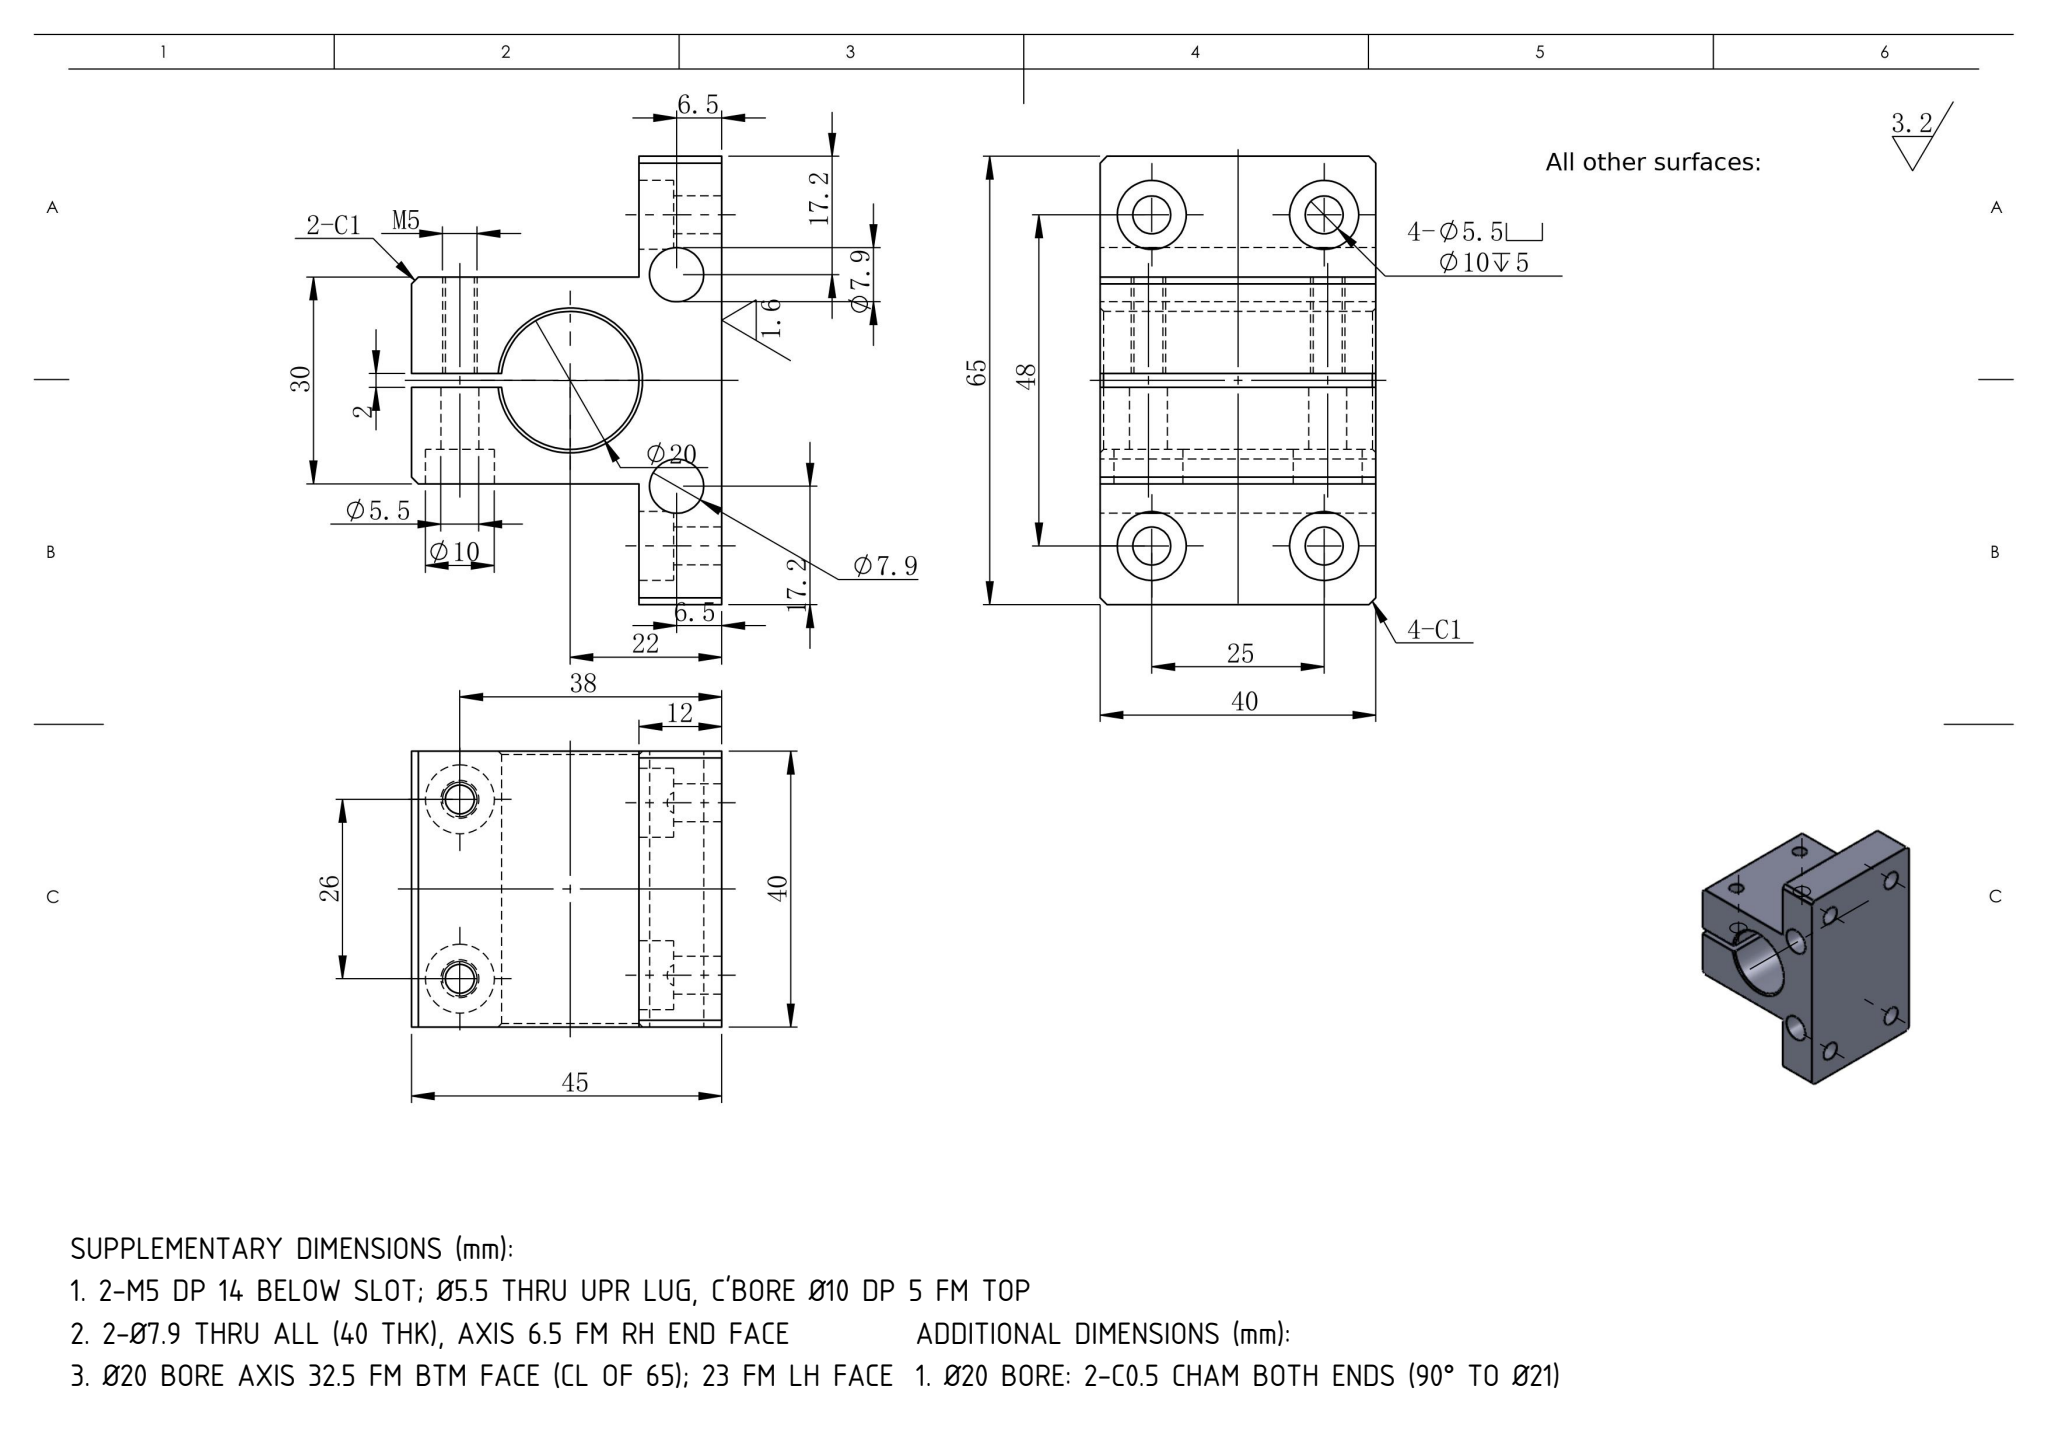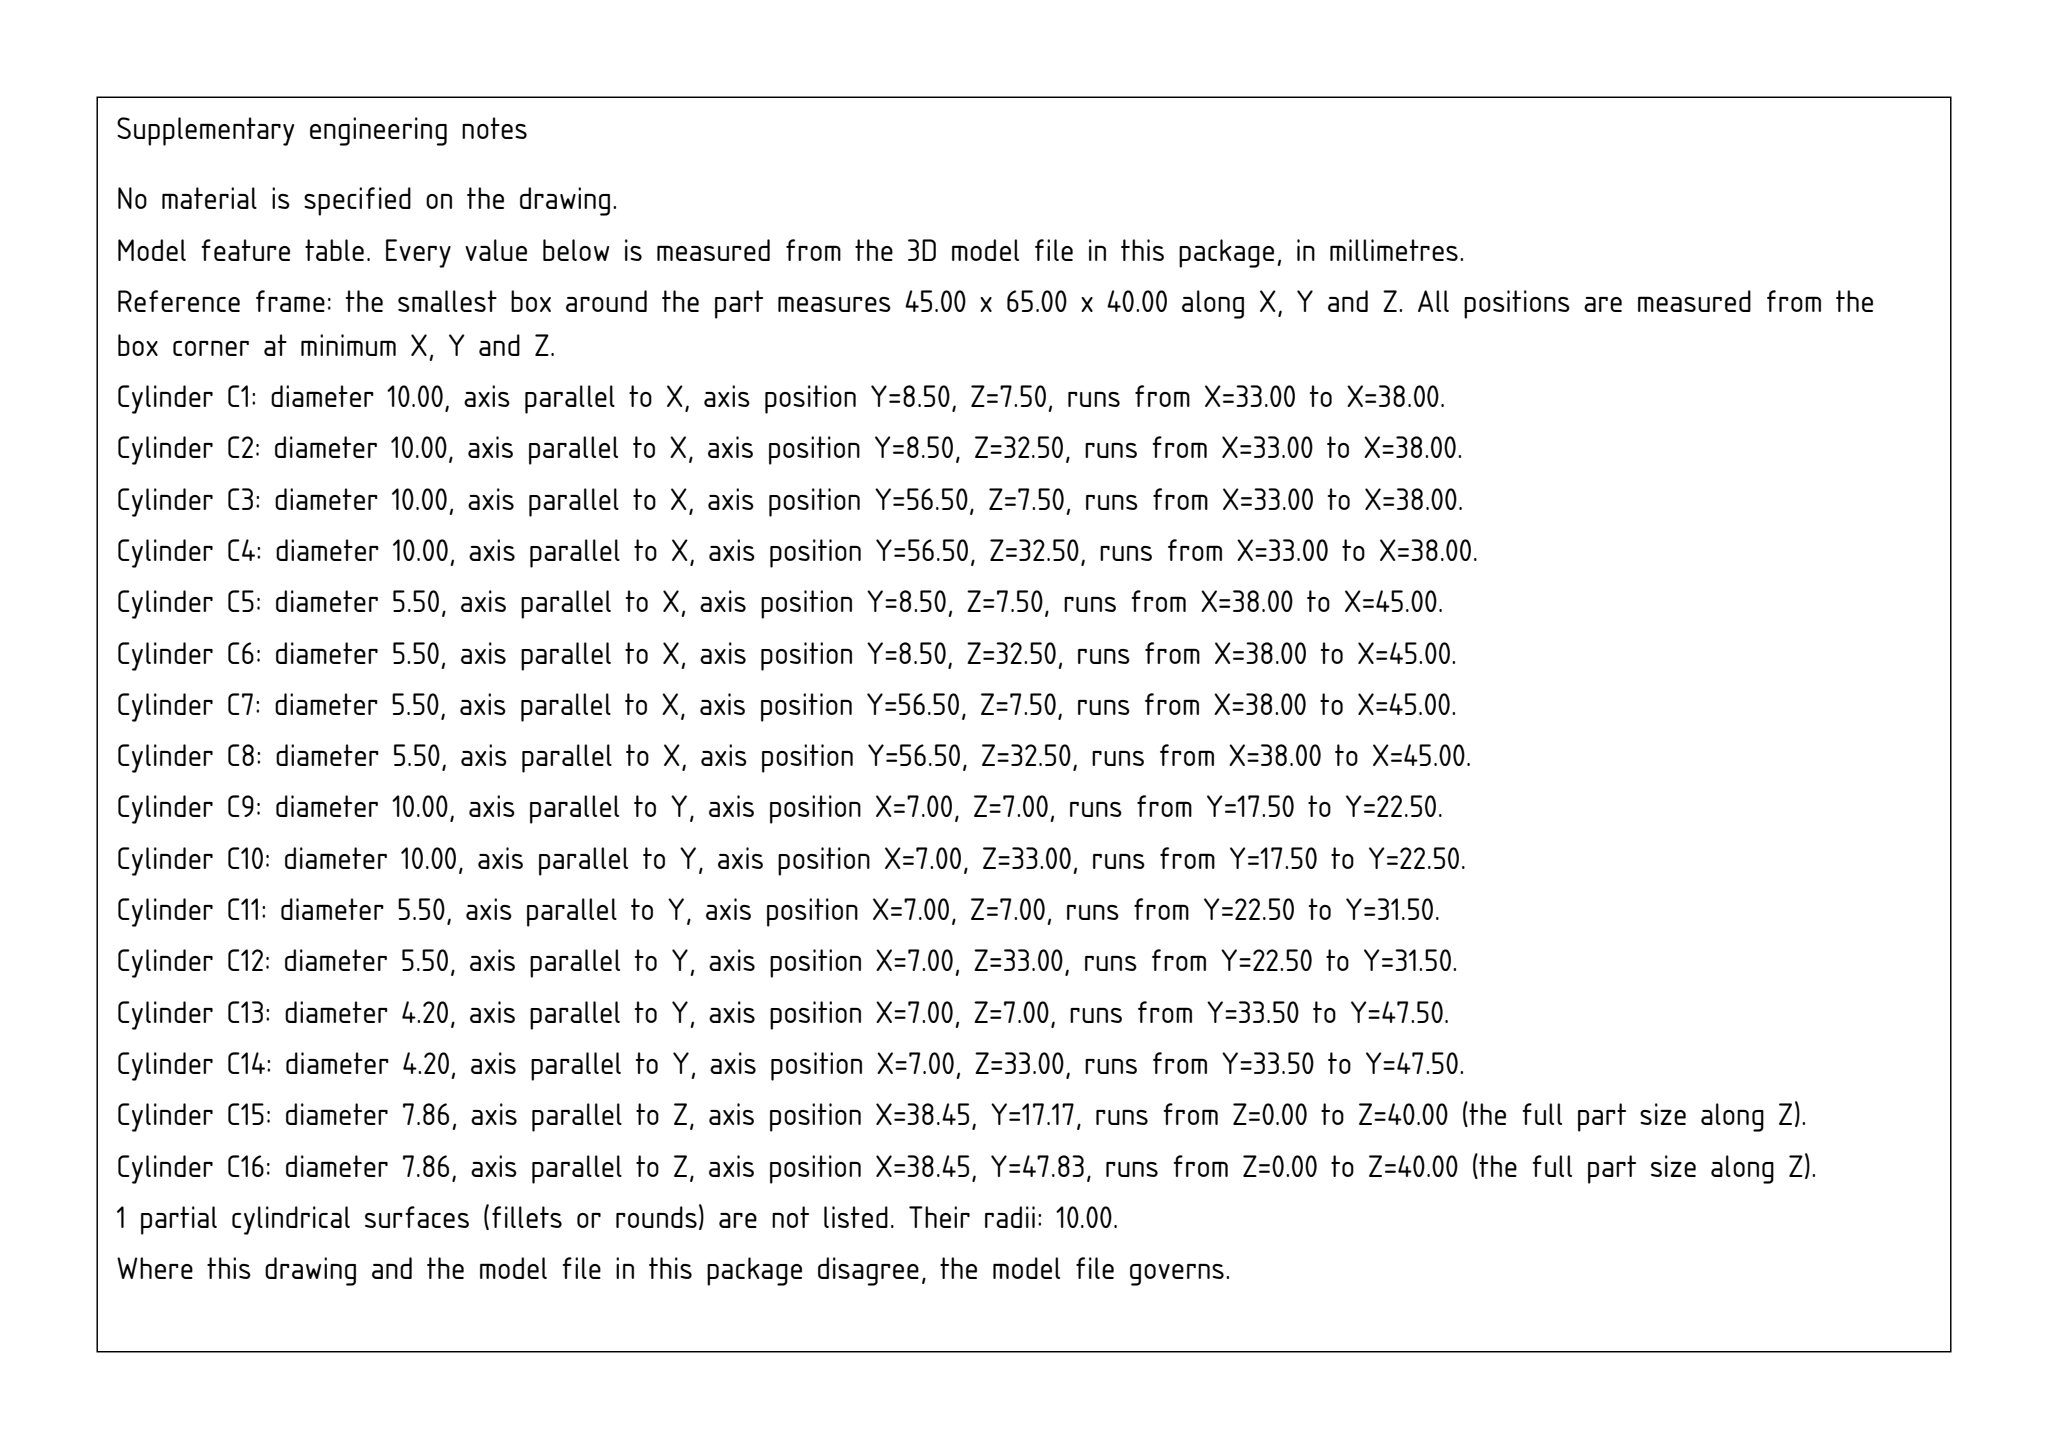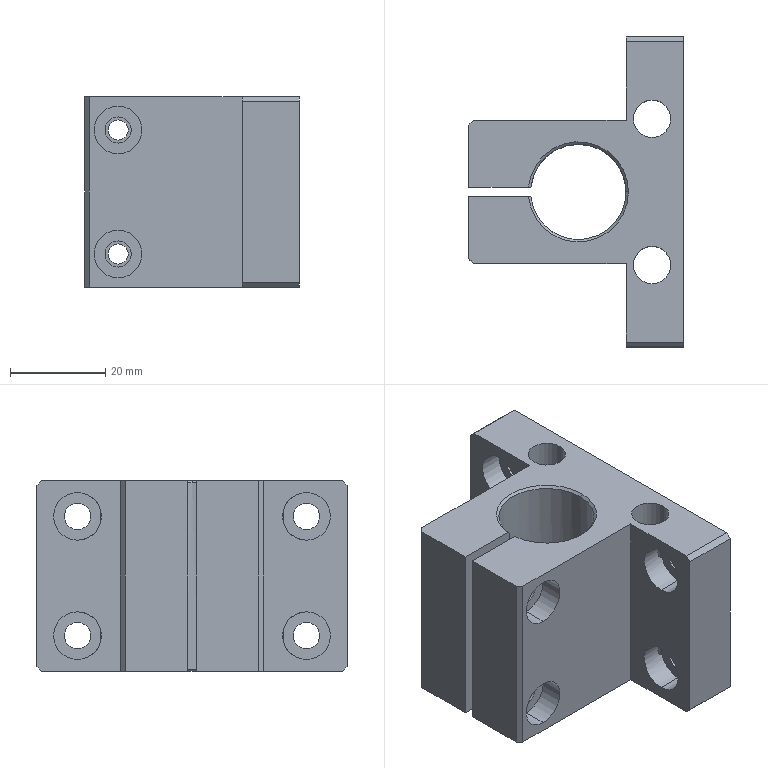Part | SolidWorks | mm | 1 solid | 61 faces | box 45 x 65 x 40 mm | volume 49401 mm3 | cylinder 33 | plane 25 | cone 3 | commonest cylinder face diameters 10 x12 5.5 x12 7.853 x4 4.2 x4 20 x1
build123d program:
from build123d import *

# Parameters (mm, degrees)
BOSS_EXTRUDE1_DEPTH                             = 40
HOLE1_D                                         = 20
SKETCH4_W                                       = 20
SKETCH4_H                                       = 2
CUT_EXTRUDE1_DEPTH                              = 69.42
CHAMFER1_SIZE                                   = 1
M5_HEX_SOCKET_HEAD_CAP_SCREW_CBORE1_D           = 5.5
M5_HEX_SOCKET_HEAD_CAP_SCREW_CBORE1_DEPTH       = 14
M5_HEX_SOCKET_HEAD_CAP_SCREW_CBORE1_CBORE_D     = 10
M5_HEX_SOCKET_HEAD_CAP_SCREW_CBORE1_CBORE_DEPTH = 5
M5_TAPPED_HOLE1_D                               = 4.2
CHAMFER2_SIZE                                   = 0.5
M5_HEX_SOCKET_HEAD_CAP_SCREW_CBORE2_D           = 5.5
M5_HEX_SOCKET_HEAD_CAP_SCREW_CBORE2_CBORE_D     = 10
M5_HEX_SOCKET_HEAD_CAP_SCREW_CBORE2_CBORE_DEPTH = 5
SKETCH13_R                                      = 3.927
CUT_EXTRUDE2_DEPTH                              = 65


with BuildPart() as part:
    # Sketch1 → Boss-Extrude1 (new body)
    with BuildSketch(Plane.XY):
        Polygon((0, -15), (0, 15), (33, 15), (33, 32.5), (45, 32.5), (45, -32.5), (33, -32.5), (33, -15), align=None)
    extrude(amount=BOSS_EXTRUDE1_DEPTH)

    # Hole1 (through all)
    with Locations(Plane(origin=(0, 0, 0), x_dir=(-1, 0, 0), z_dir=(0, 0, -1))):
        with Locations((-23, 0)):
            Hole(HOLE1_D / 2)

    # Sketch4 → Cut-Extrude1 (cut, through all)
    with BuildSketch(Plane(origin=(0, 0, 0), x_dir=(-1, 0, 0), z_dir=(0, 0, -1))):
        with Locations((-10, 0)):
            Rectangle(SKETCH4_W, SKETCH4_H)
    extrude(amount=-CUT_EXTRUDE1_DEPTH, mode=Mode.SUBTRACT)

    # Chamfer1
    chamfer1_edges = [part.edges().sort_by_distance(p)[0] for p in [
        (0, -15, 20),
        (0, 15, 20),
        (39, -32.5, 40),
        (39, 32.5, 40),
        (39, 32.5, 0),
        (39, -32.5, 0),
    ]]
    chamfer(chamfer1_edges, length=CHAMFER1_SIZE)

    # M5 Hex Socket Head Cap Screw CBORE1
    with Locations(Plane.XZ.offset(15)):
        with Locations((7, 33), (7, 7)):
            CounterBoreHole(M5_HEX_SOCKET_HEAD_CAP_SCREW_CBORE1_D / 2, M5_HEX_SOCKET_HEAD_CAP_SCREW_CBORE1_CBORE_D / 2, M5_HEX_SOCKET_HEAD_CAP_SCREW_CBORE1_CBORE_DEPTH, depth=M5_HEX_SOCKET_HEAD_CAP_SCREW_CBORE1_DEPTH)

    # M5 Tapped Hole1 (through all)
    with Locations(Plane.XZ.offset(-1)):
        with Locations((7, 33), (7, 7)):
            Hole(M5_TAPPED_HOLE1_D / 2)

    # Chamfer2
    chamfer2_edges = [part.edges().sort_by_distance(p)[0] for p in [
        (23.501, 9.987, 0),
        (23.501, -9.987, 40),
    ]]
    chamfer(chamfer2_edges, length=CHAMFER2_SIZE)

    # M5 Hex Socket Head Cap Screw CBORE2 (through all)
    with Locations(Plane.ZY.offset(-33)):
        with Locations((7.5, 24), (32.5, 24), (32.5, -24), (7.5, -24)):
            CounterBoreHole(M5_HEX_SOCKET_HEAD_CAP_SCREW_CBORE2_D / 2, M5_HEX_SOCKET_HEAD_CAP_SCREW_CBORE2_CBORE_D / 2, M5_HEX_SOCKET_HEAD_CAP_SCREW_CBORE2_CBORE_DEPTH)

    # Sketch13 → Cut-Extrude2 (cut)
    with BuildSketch(Plane(origin=(0, 0, 0), x_dir=(-1, 0, 0), z_dir=(0, 0, -1))):
        with Locations((-38.45, 15.33)):
            Circle(SKETCH13_R)
        with Locations((-38.45, -15.33)):
            Circle(SKETCH13_R)
    extrude(amount=-CUT_EXTRUDE2_DEPTH, mode=Mode.SUBTRACT)


solid = part.part